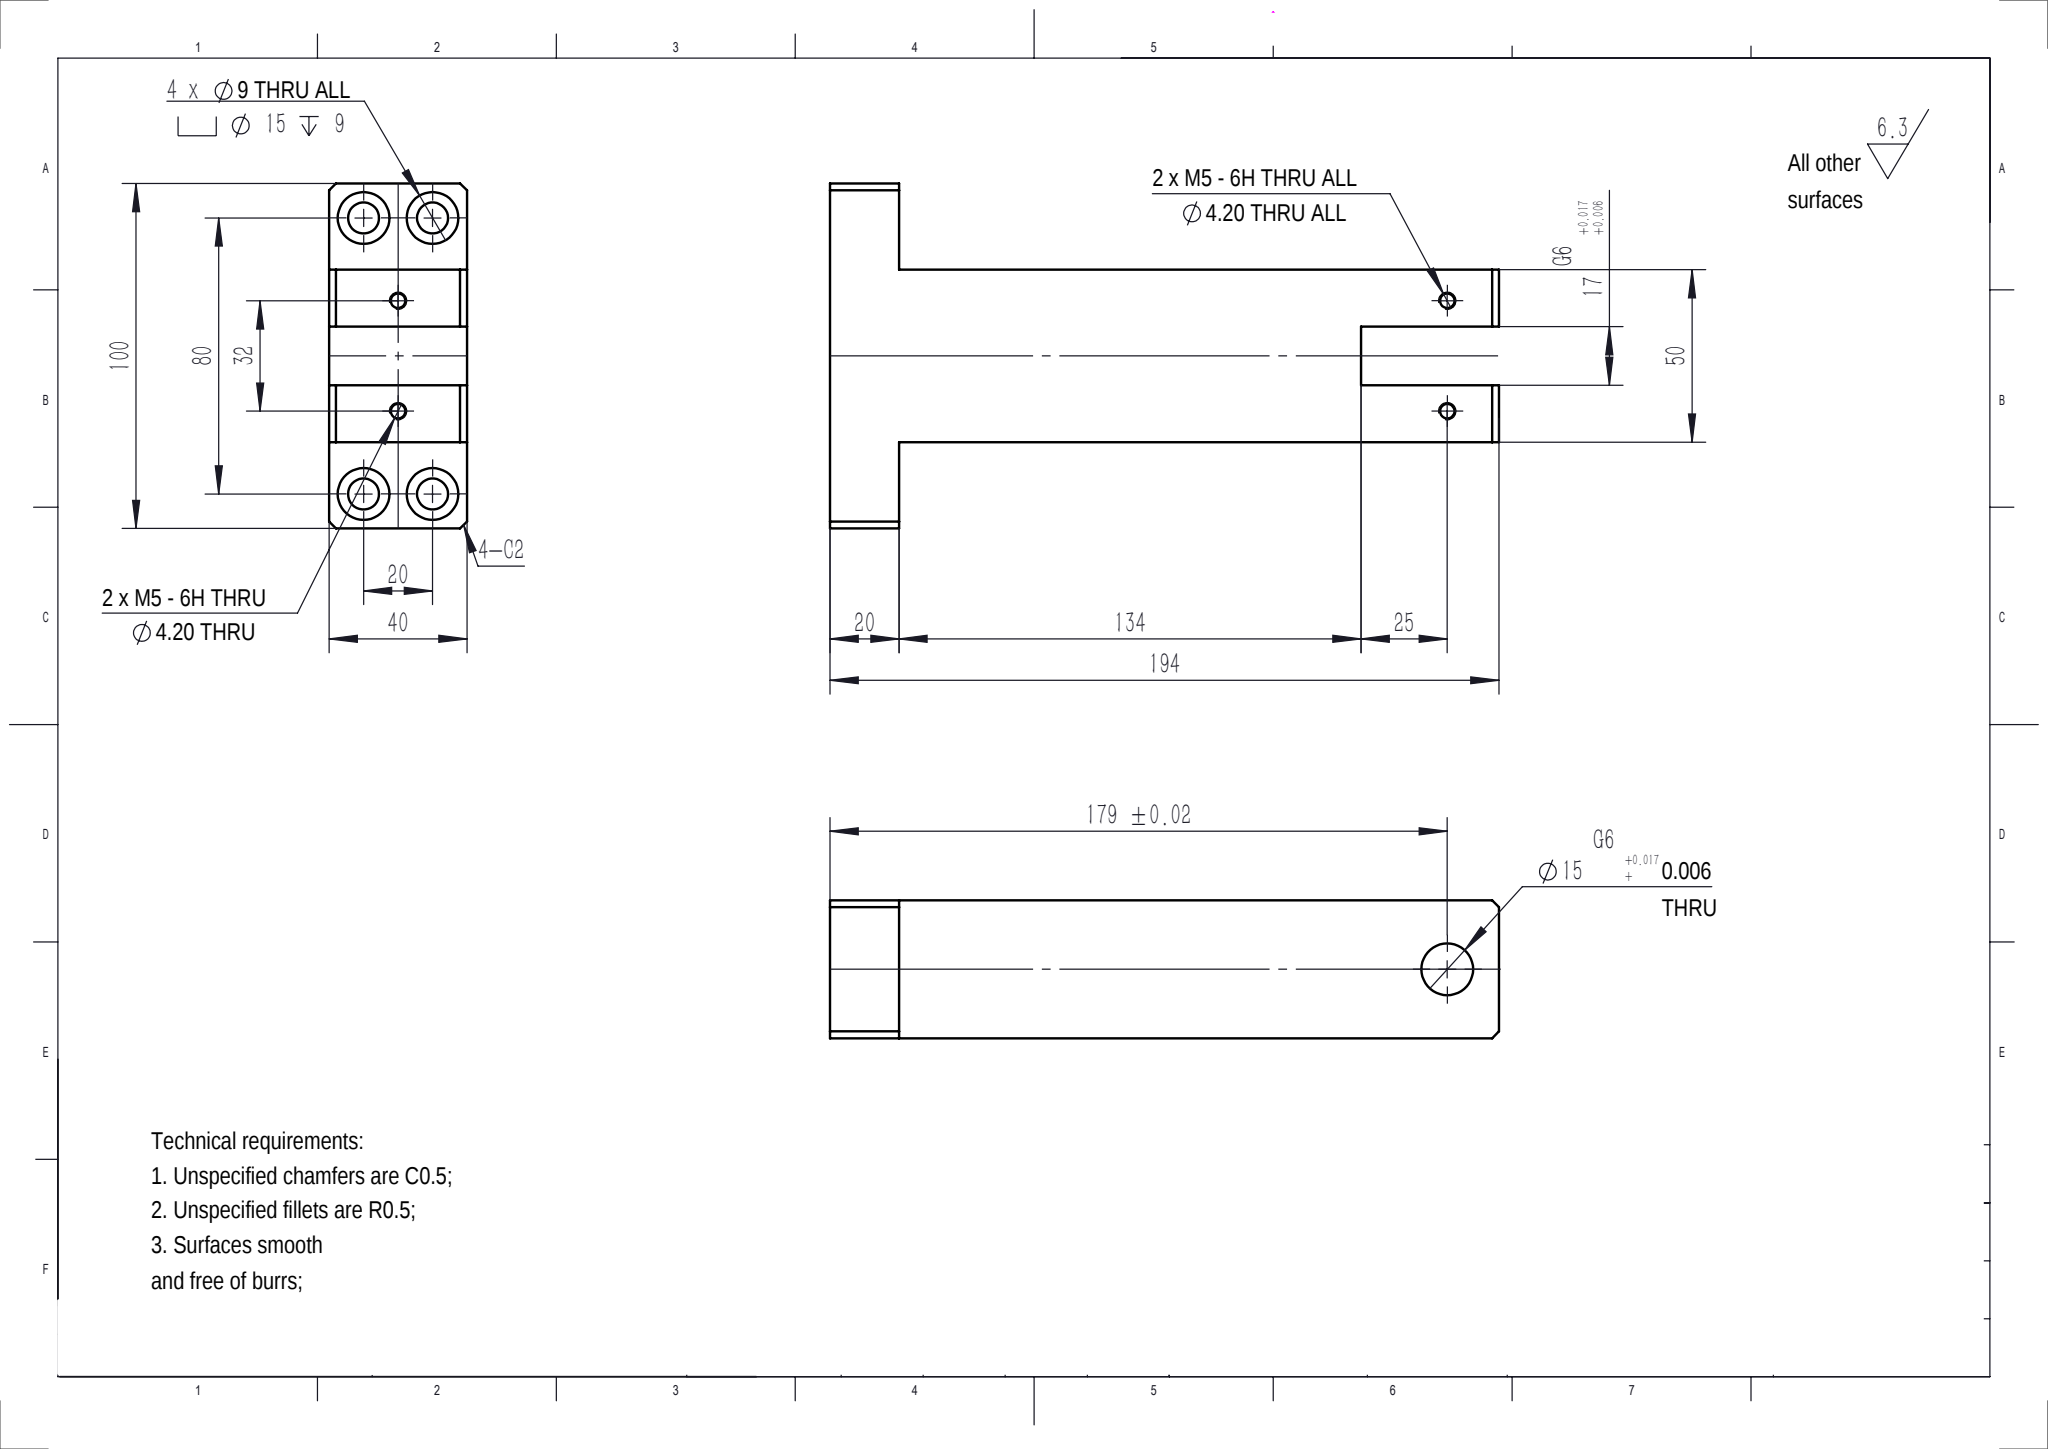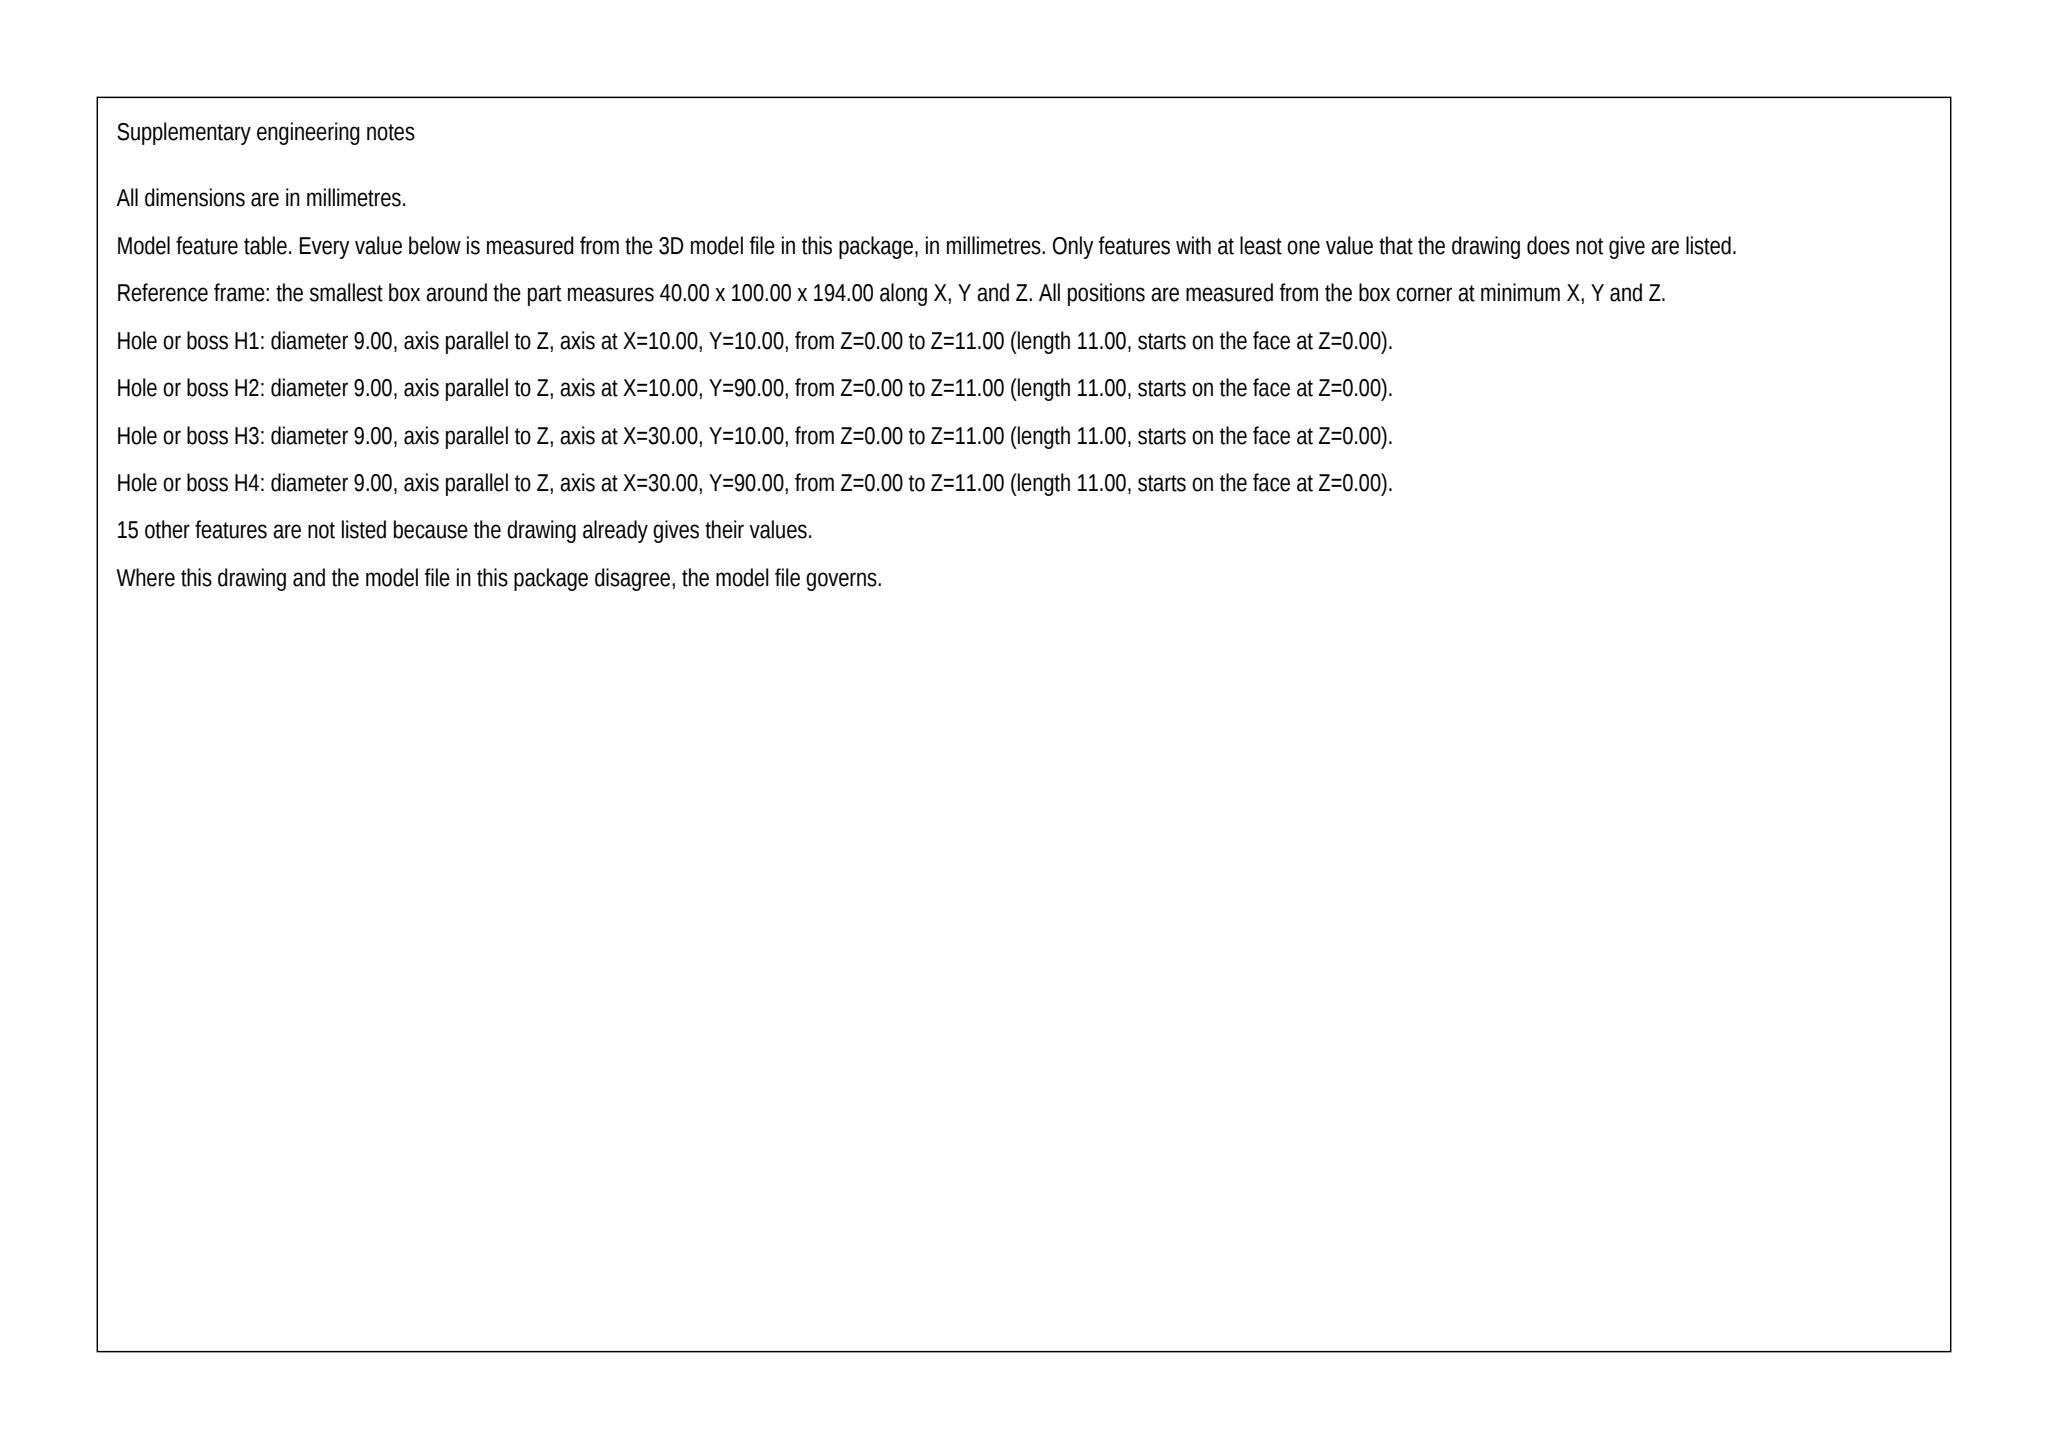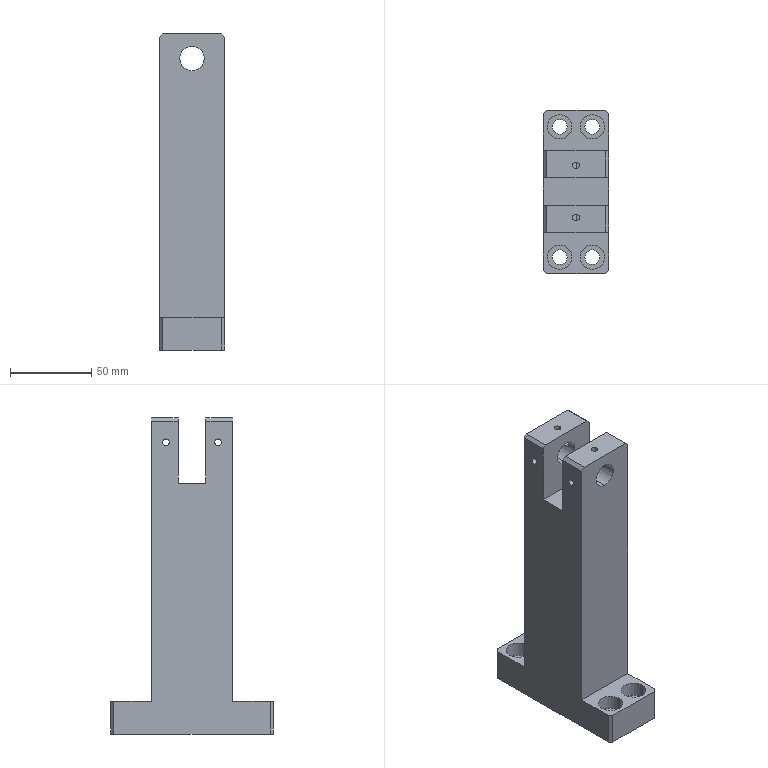Part | SolidWorks | mm | 1 solid | 58 faces | box 40 x 100 x 194 mm | volume 384609 mm3 | cylinder 32 | plane 26 | commonest cylinder face diameters 4.2 x12 15 x12 9 x8
build123d program:
from build123d import *

# Parameters (mm, degrees)
BOSS_EXTRUDE1_DEPTH                               = 40
HOLE_SIZE_ACCORDING_TO_HEX_SOCKET_HEA_D           = 9
HOLE_SIZE_ACCORDING_TO_HEX_SOCKET_HEA_CBORE_D     = 15
HOLE_SIZE_ACCORDING_TO_HEX_SOCKET_HEA_CBORE_DEPTH = 9
SKETCH5_W                                         = 40
SKETCH5_H                                         = 17
CUT_EXTRUDE1_DEPTH                                = 212.804
SKETCH6_R                                         = 7.5
CUT_EXTRUDE2_DEPTH                                = 212.804
M5_TAPPED_HOLE1_D                                 = 4.2
M5_TAPPED_HOLE2_REACH                             = 213.804
M5_TAPPED_HOLE2_BORE_R                            = 2.1
CHAMFER1_SIZE                                     = 2


with BuildPart() as part:
    # Sketch1 → Boss-Extrude1 (new body)
    with BuildSketch(Plane(origin=(0, 0, 0), x_dir=(0, 0, -1), z_dir=(1, 0, 0))):
        Polygon((0, 0), (174, 0), (174, 25), (194, 25), (194, -75), (174, -75), (174, -50), (0, -50), align=None)
    extrude(amount=BOSS_EXTRUDE1_DEPTH)

    # Hole Size _ according to_ Hex Socket Hea (through all)
    with Locations(Plane.XY.offset(-174)):
        with Locations((10, 15), (10, -65), (30, 15), (30, -65)):
            CounterBoreHole(HOLE_SIZE_ACCORDING_TO_HEX_SOCKET_HEA_D / 2, HOLE_SIZE_ACCORDING_TO_HEX_SOCKET_HEA_CBORE_D / 2, HOLE_SIZE_ACCORDING_TO_HEX_SOCKET_HEA_CBORE_DEPTH)

    # Sketch5 → Cut-Extrude1 (cut, through all)
    with BuildSketch(Plane(origin=(40, 0, 0), x_dir=(0, 0, -1), z_dir=(1, 0, 0))):
        with Locations((20, -25)):
            Rectangle(SKETCH5_W, SKETCH5_H)
    extrude(amount=-CUT_EXTRUDE1_DEPTH, mode=Mode.SUBTRACT)

    # Sketch6 → Cut-Extrude2 (cut, through all)
    with BuildSketch(Plane.XZ.offset(50)):
        with Locations(Location((20, -15, 0), (0, 0, 270))):
            Circle(SKETCH6_R)
    extrude(amount=-CUT_EXTRUDE2_DEPTH, mode=Mode.SUBTRACT)

    # M5 Tapped Hole1 (through all)
    with Locations(Plane(origin=(40, 0, 0), x_dir=(0, 0, -1), z_dir=(1, 0, 0))):
        with Locations((15, -9), (15, -41)):
            Hole(M5_TAPPED_HOLE1_D / 2)

    # M5 Tapped Hole2 bore → M5 Tapped Hole2 (cut, up to next)
    with BuildSketch(Plane.XY, mode=Mode.PRIVATE) as m5_tapped_hole2_sk1:
        with Locations((20, -9)):
            Circle(M5_TAPPED_HOLE2_BORE_R)
    m5_tapped_hole2_tool1 = extrude(m5_tapped_hole2_sk1.sketch, amount=-M5_TAPPED_HOLE2_REACH, mode=Mode.PRIVATE) & part.part
    # M5 Tapped Hole2 bore → M5 Tapped Hole2 (cut, up to next)
    with BuildSketch(Plane.XY, mode=Mode.PRIVATE) as m5_tapped_hole2_sk2:
        with Locations((20, -41)):
            Circle(M5_TAPPED_HOLE2_BORE_R)
    m5_tapped_hole2_tool2 = extrude(m5_tapped_hole2_sk2.sketch, amount=-M5_TAPPED_HOLE2_REACH, mode=Mode.PRIVATE) & part.part
    add(m5_tapped_hole2_tool1.solids().sort_by_distance((20, -9, 0))[0], mode=Mode.SUBTRACT)
    add(m5_tapped_hole2_tool2.solids().sort_by_distance((20, -41, 0))[0], mode=Mode.SUBTRACT)

    # Chamfer1
    chamfer1_edges = [part.edges().sort_by_distance(p)[0] for p in [
        (0, -8.25, 0),
        (40, -75, -184),
        (40, 25, -184),
        (40, -8.25, 0),
        (0, -41.75, 0),
        (40, -41.75, 0),
        (0, 25, -184),
        (0, -75, -184),
    ]]
    chamfer(chamfer1_edges, length=CHAMFER1_SIZE)


solid = part.part